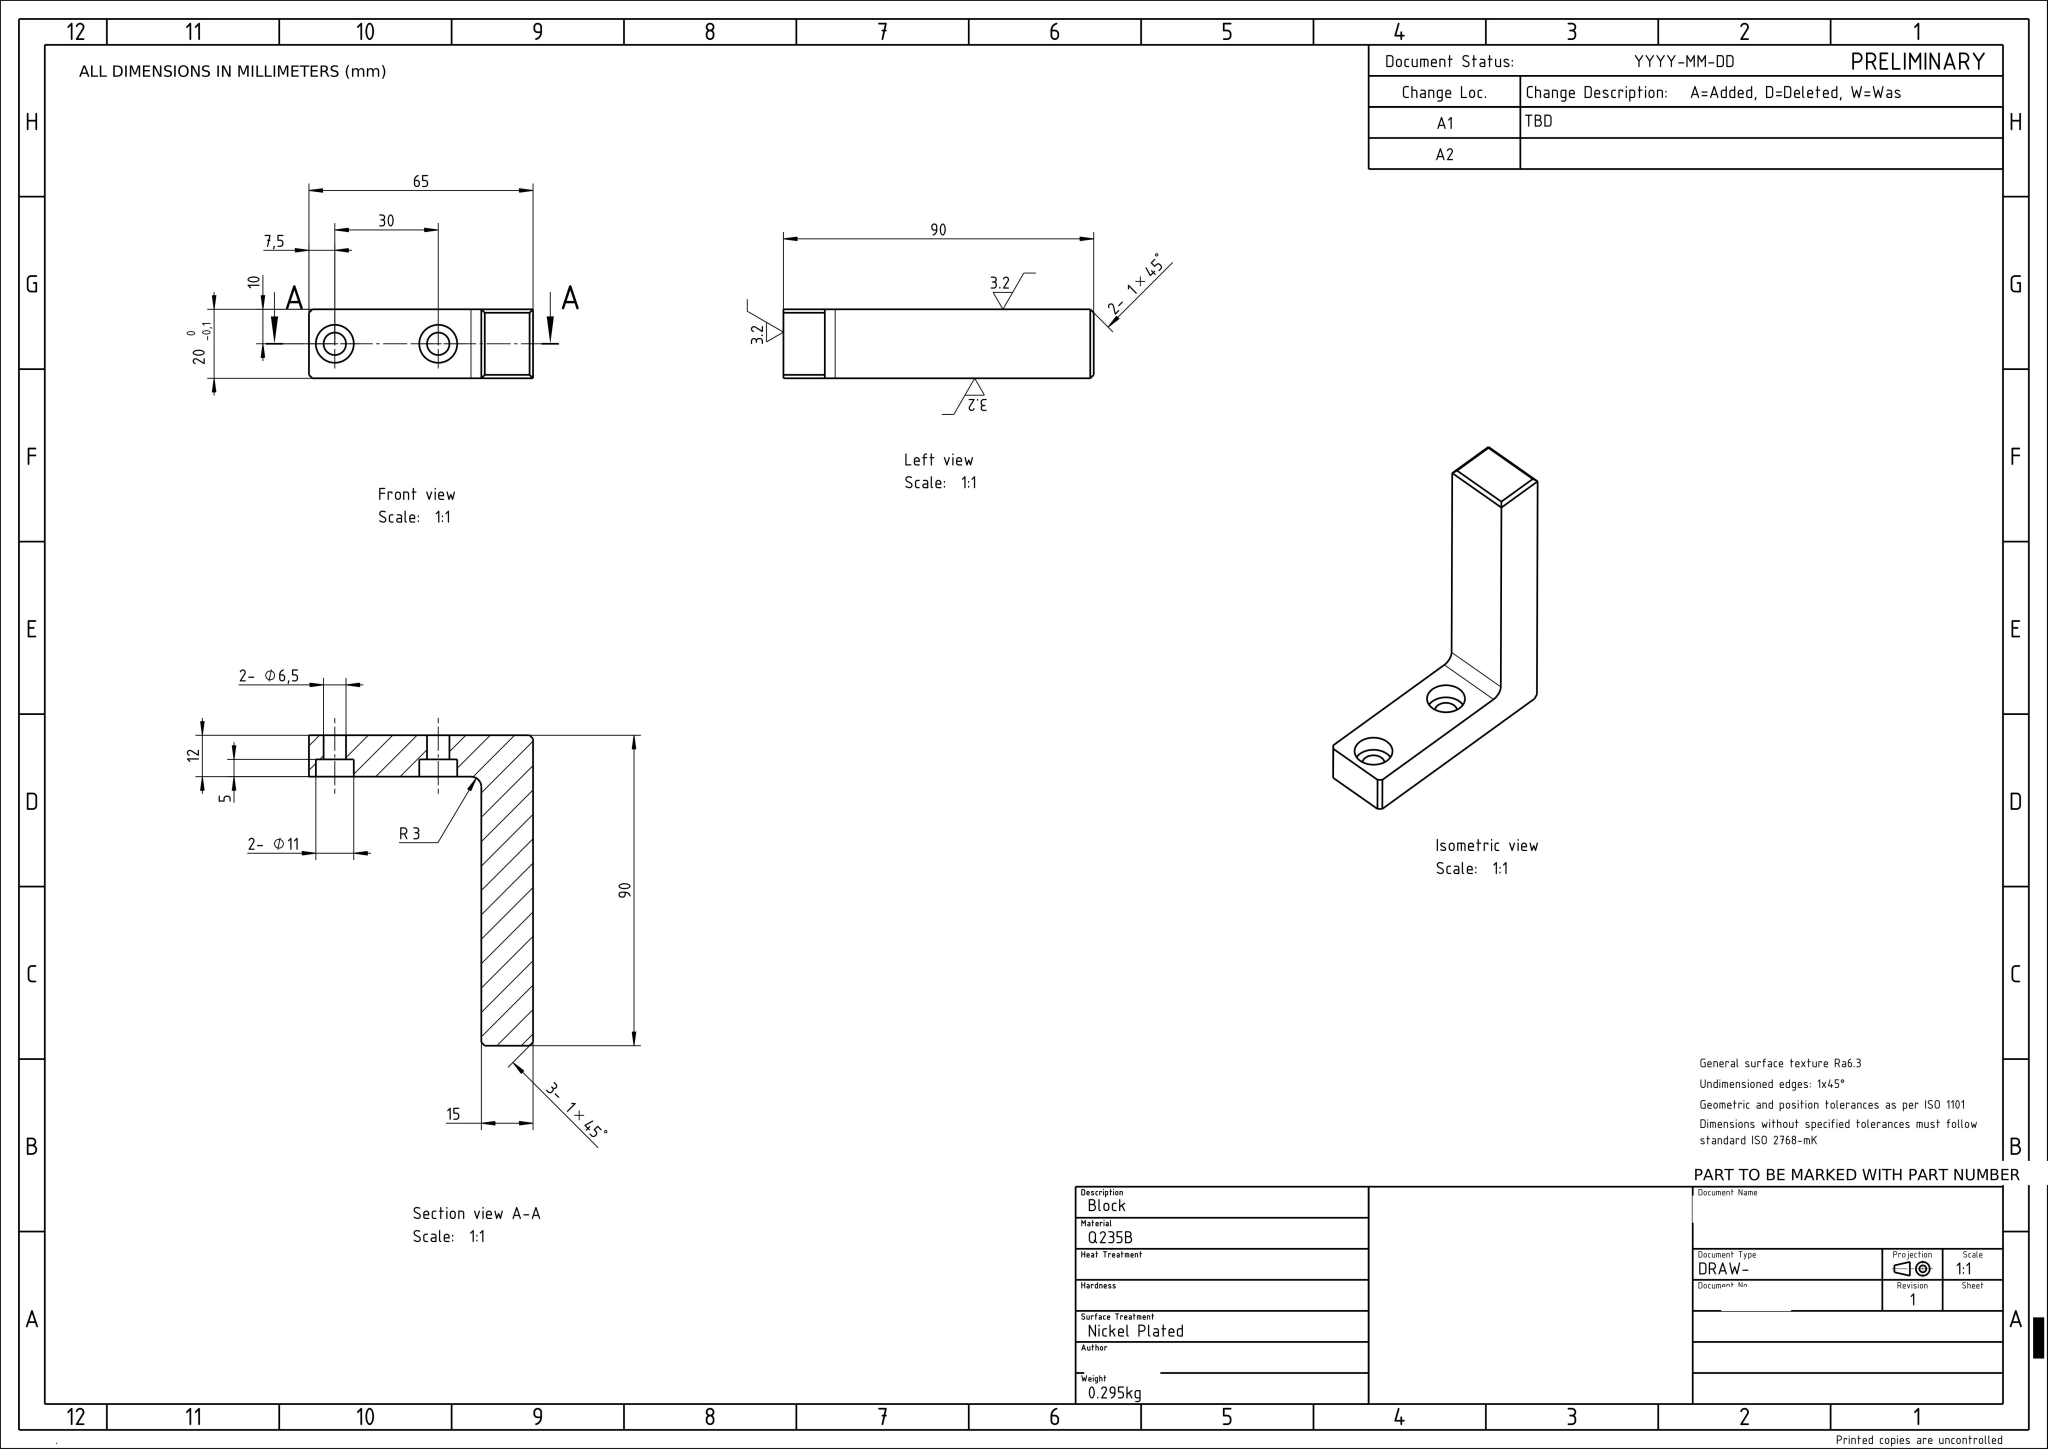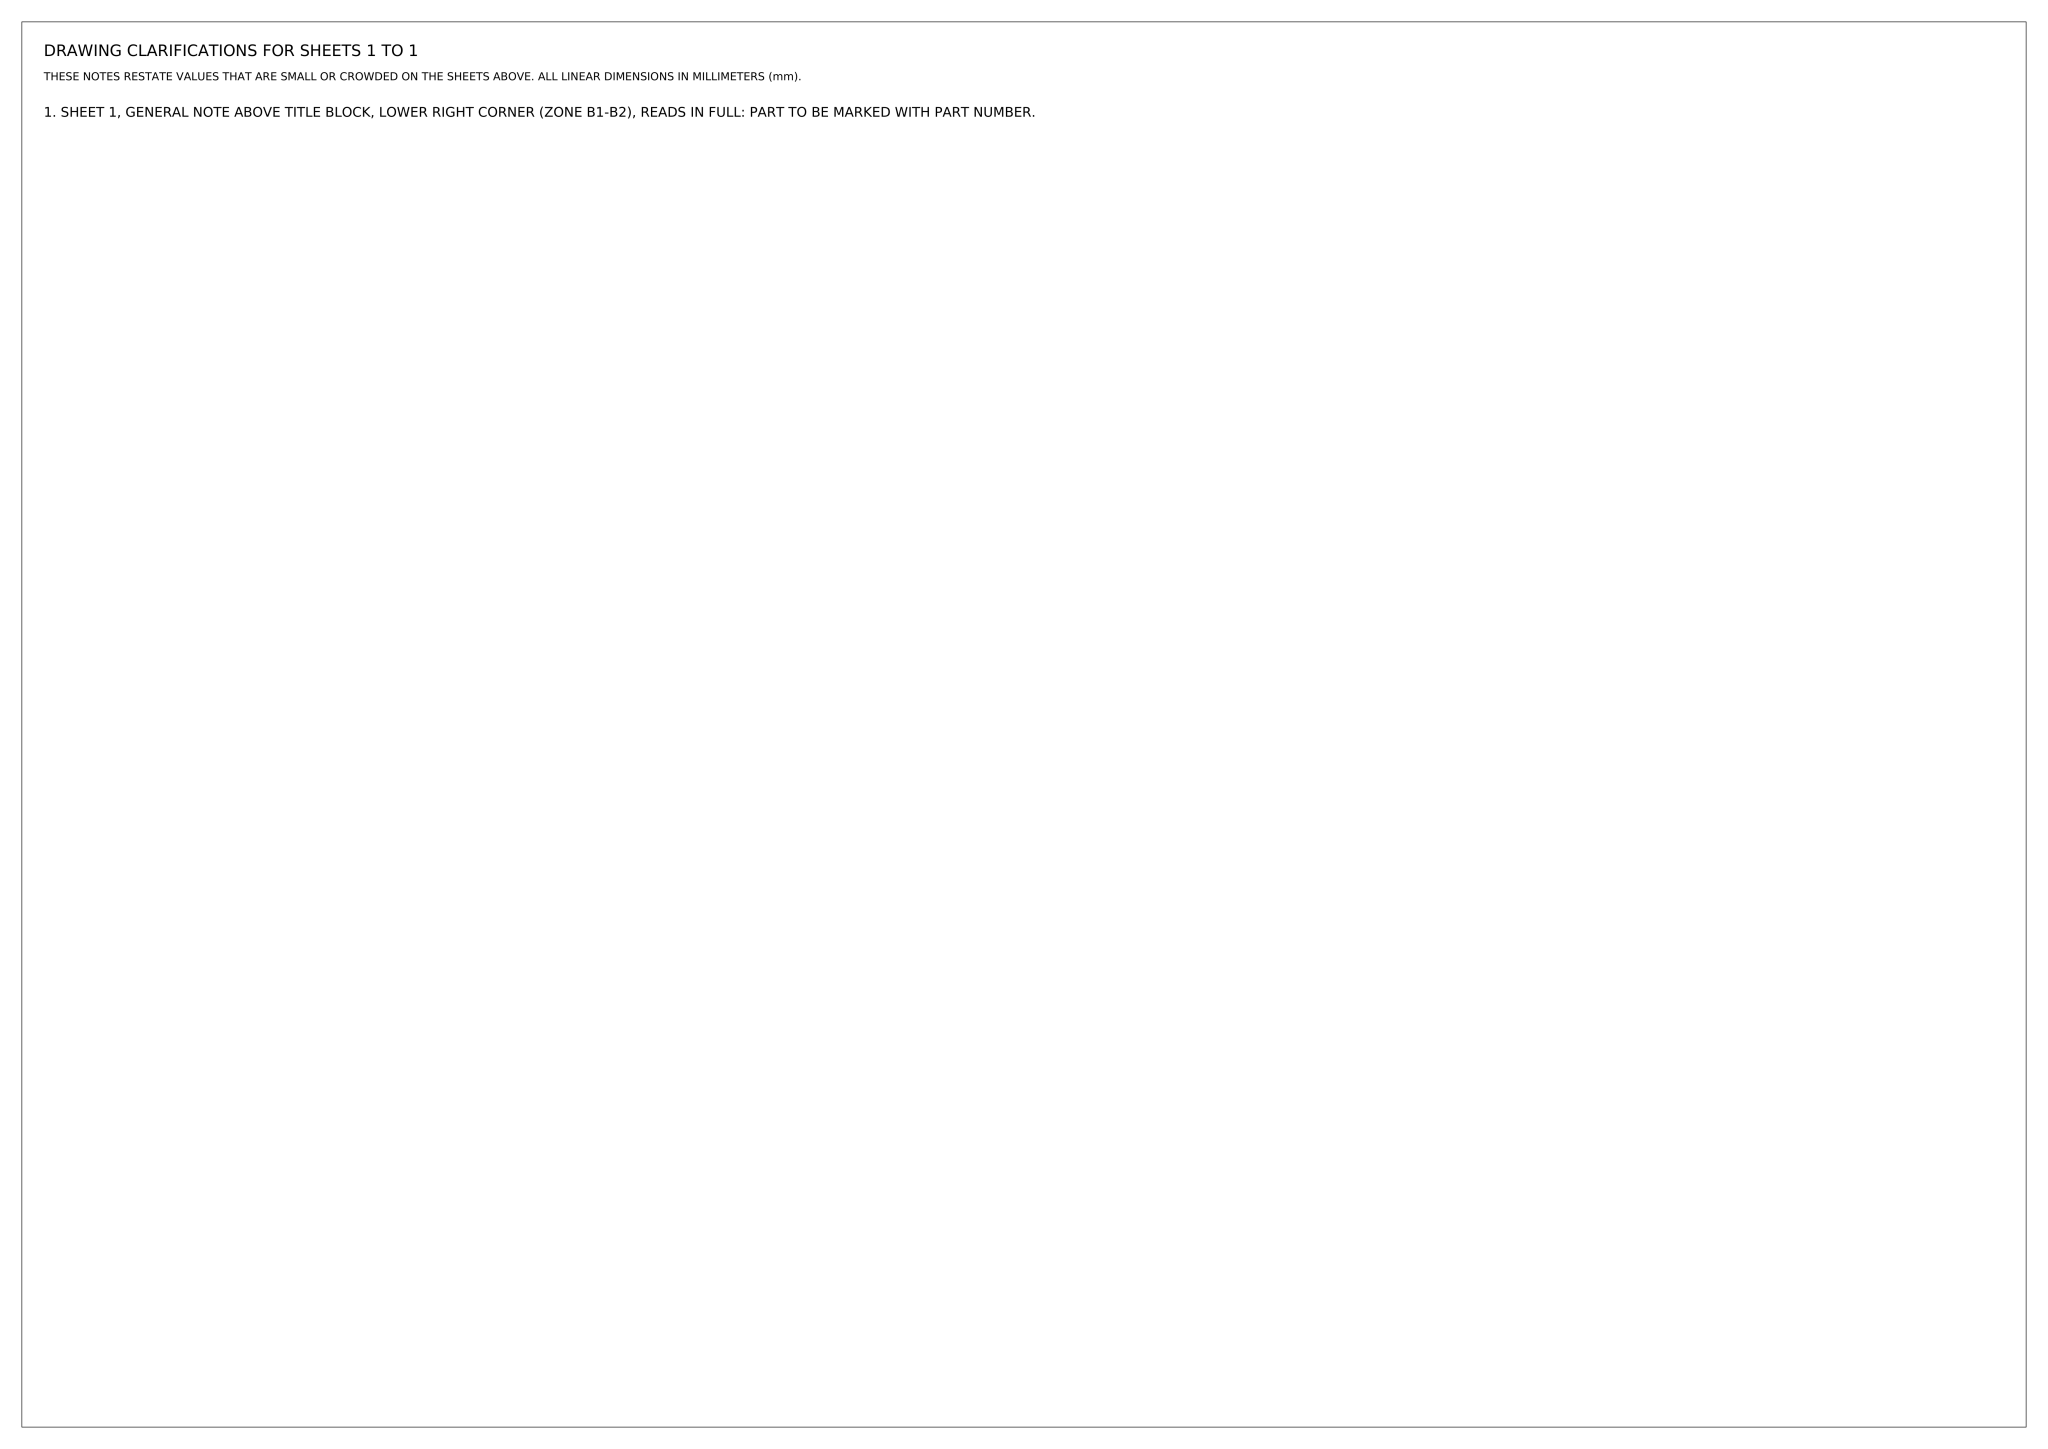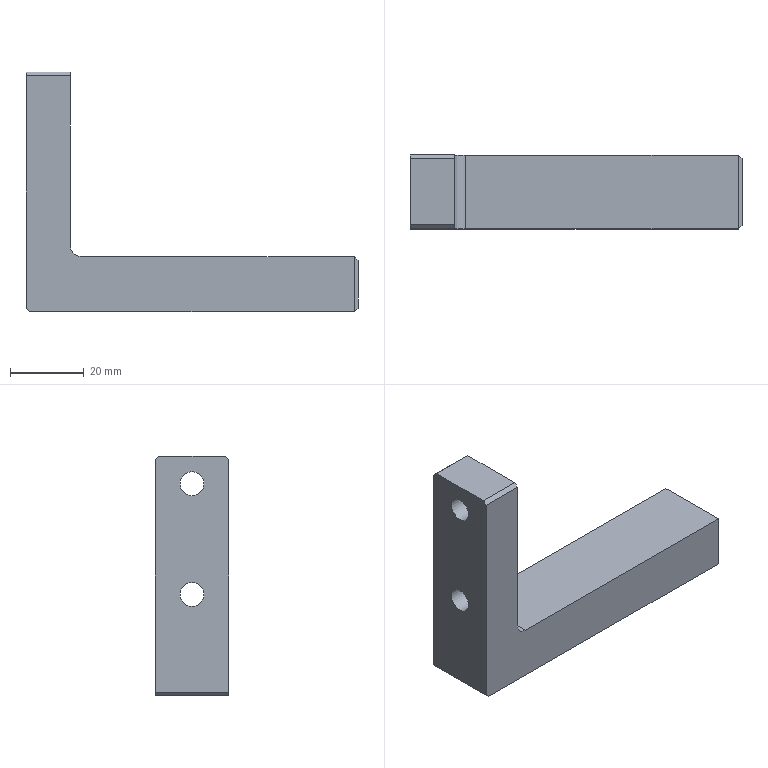Part | NX | mm | 1 solid | 22 faces | box 90 x 20 x 65 mm | volume 37568 mm3 | plane 17 | cylinder 5 | commonest cylinder face diameters 6.5 x2 11 x2 6 x1
STEP:
#1=CARTESIAN_POINT('',(0.,0.,0.));
#2=DIRECTION('',(0.,0.,1.));
#3=DIRECTION('',(1.,0.,0.));
#4=AXIS2_PLACEMENT_3D('',#1,#2,#3);
#5=(LENGTH_UNIT()NAMED_UNIT(*)SI_UNIT(.MILLI.,.METRE.));
#6=UNCERTAINTY_MEASURE_WITH_UNIT(LENGTH_MEASURE(0.00002),#5,'','');
#7=(NAMED_UNIT(*)PLANE_ANGLE_UNIT()SI_UNIT($,.RADIAN.));
#8=PLANE_ANGLE_MEASURE_WITH_UNIT(PLANE_ANGLE_MEASURE(0.01745),#7);
#9=DIMENSIONAL_EXPONENTS(0.,0.,0.,0.,0.,0.,0.);
#10=(CONVERSION_BASED_UNIT('',#8)NAMED_UNIT(#9)PLANE_ANGLE_UNIT());
#11=(NAMED_UNIT(*)SI_UNIT($,.STERADIAN.)SOLID_ANGLE_UNIT());
#12=(GEOMETRIC_REPRESENTATION_CONTEXT(3)GLOBAL_UNCERTAINTY_ASSIGNED_CONTEXT((#6))GLOBAL_UNIT_ASSIGNED_CONTEXT((#5,#10,#11))REPRESENTATION_CONTEXT('',''));
#13=SHAPE_REPRESENTATION('',(#4),#12);
#14=CARTESIAN_POINT('',(0.,-0.,54.25));
#15=VERTEX_POINT('',#14);
#16=CARTESIAN_POINT('',(0.,-0.,57.5));
#17=DIRECTION('',(1.,0.,0.));
#18=DIRECTION('',(0.,0.,-1.));
#19=AXIS2_PLACEMENT_3D('',#16,#17,#18);
#20=CIRCLE('',#19,3.25);
#21=EDGE_CURVE('',#15,#15,#20,.T.);
#22=ORIENTED_EDGE('',*,*,#21,.T.);
#23=EDGE_LOOP('',(#22));
#24=FACE_BOUND('',#23,.T.);
#25=CARTESIAN_POINT('',(0.,-0.,24.25));
#26=VERTEX_POINT('',#25);
#27=CARTESIAN_POINT('',(0.,-0.,27.5));
#28=DIRECTION('',(1.,0.,0.));
#29=DIRECTION('',(0.,0.,-1.));
#30=AXIS2_PLACEMENT_3D('',#27,#28,#29);
#31=CIRCLE('',#30,3.25);
#32=EDGE_CURVE('',#26,#26,#31,.T.);
#33=ORIENTED_EDGE('',*,*,#32,.T.);
#34=EDGE_LOOP('',(#33));
#35=FACE_BOUND('',#34,.T.);
#36=CARTESIAN_POINT('',(0.,10.,64.));
#37=VERTEX_POINT('',#36);
#38=CARTESIAN_POINT('',(0.,10.,1.));
#39=VERTEX_POINT('',#38);
#40=CARTESIAN_POINT('',(0.,10.,15.));
#41=DIRECTION('',(0.,0.,-1.));
#42=VECTOR('',#41,1.);
#43=LINE('',#40,#42);
#44=EDGE_CURVE('',#37,#39,#43,.T.);
#45=ORIENTED_EDGE('',*,*,#44,.T.);
#46=CARTESIAN_POINT('',(0.,-10.,1.));
#47=VERTEX_POINT('',#46);
#48=CARTESIAN_POINT('',(0.,10.,1.));
#49=DIRECTION('',(0.,-1.,0.));
#50=VECTOR('',#49,1.);
#51=LINE('',#48,#50);
#52=EDGE_CURVE('',#39,#47,#51,.T.);
#53=ORIENTED_EDGE('',*,*,#52,.T.);
#54=CARTESIAN_POINT('',(0.,-10.,64.));
#55=VERTEX_POINT('',#54);
#56=CARTESIAN_POINT('',(0.,-10.,15.));
#57=DIRECTION('',(0.,0.,-1.));
#58=VECTOR('',#57,1.);
#59=LINE('',#56,#58);
#60=EDGE_CURVE('',#55,#47,#59,.T.);
#61=ORIENTED_EDGE('',*,*,#60,.F.);
#62=CARTESIAN_POINT('',(0.,-9.,65.));
#63=VERTEX_POINT('',#62);
#64=CARTESIAN_POINT('',(0.,-9.,65.));
#65=DIRECTION('',(0.,0.7071,0.7071));
#66=VECTOR('',#65,1.);
#67=LINE('',#64,#66);
#68=EDGE_CURVE('',#55,#63,#67,.T.);
#69=ORIENTED_EDGE('',*,*,#68,.T.);
#70=CARTESIAN_POINT('',(0.,9.,65.));
#71=VERTEX_POINT('',#70);
#72=CARTESIAN_POINT('',(0.,-10.,65.));
#73=DIRECTION('',(0.,1.,0.));
#74=VECTOR('',#73,1.);
#75=LINE('',#72,#74);
#76=EDGE_CURVE('',#63,#71,#75,.T.);
#77=ORIENTED_EDGE('',*,*,#76,.T.);
#78=CARTESIAN_POINT('',(0.,10.,64.));
#79=DIRECTION('',(0.,0.7071,-0.7071));
#80=VECTOR('',#79,1.);
#81=LINE('',#78,#80);
#82=EDGE_CURVE('',#71,#37,#81,.T.);
#83=ORIENTED_EDGE('',*,*,#82,.T.);
#84=EDGE_LOOP('',(#45,#53,#61,#69,#77,#83));
#85=FACE_BOUND('',#84,.T.);
#86=CARTESIAN_POINT('',(0.,10.,15.));
#87=DIRECTION('',(1.,0.,0.));
#88=DIRECTION('',(0.,0.,-1.));
#89=AXIS2_PLACEMENT_3D('',#86,#87,#88);
#90=PLANE('',#89);
#91=ADVANCED_FACE('',(#24,#35,#85),#90,.F.);
#92=ORIENTED_EDGE('',*,*,#60,.T.);
#93=CARTESIAN_POINT('',(1.,-10.,0.));
#94=VERTEX_POINT('',#93);
#95=CARTESIAN_POINT('',(0.,-10.,1.));
#96=DIRECTION('',(0.7071,0.,-0.7071));
#97=VECTOR('',#96,1.);
#98=LINE('',#95,#97);
#99=EDGE_CURVE('',#47,#94,#98,.T.);
#100=ORIENTED_EDGE('',*,*,#99,.T.);
#101=CARTESIAN_POINT('',(89.,-10.,0.));
#102=VERTEX_POINT('',#101);
#103=CARTESIAN_POINT('',(0.,-10.,0.));
#104=DIRECTION('',(1.,0.,0.));
#105=VECTOR('',#104,1.);
#106=LINE('',#103,#105);
#107=EDGE_CURVE('',#94,#102,#106,.T.);
#108=ORIENTED_EDGE('',*,*,#107,.T.);
#109=CARTESIAN_POINT('',(89.,-10.,15.));
#110=VERTEX_POINT('',#109);
#111=CARTESIAN_POINT('',(89.,-10.,15.));
#112=DIRECTION('',(0.,0.,1.));
#113=VECTOR('',#112,1.);
#114=LINE('',#111,#113);
#115=EDGE_CURVE('',#102,#110,#114,.T.);
#116=ORIENTED_EDGE('',*,*,#115,.T.);
#117=CARTESIAN_POINT('',(15.,-10.,15.));
#118=VERTEX_POINT('',#117);
#119=CARTESIAN_POINT('',(0.,-10.,15.));
#120=DIRECTION('',(1.,0.,0.));
#121=VECTOR('',#120,1.);
#122=LINE('',#119,#121);
#123=EDGE_CURVE('',#118,#110,#122,.T.);
#124=ORIENTED_EDGE('',*,*,#123,.F.);
#125=CARTESIAN_POINT('',(12.,-10.,18.));
#126=VERTEX_POINT('',#125);
#127=CARTESIAN_POINT('',(15.,-10.,18.));
#128=DIRECTION('',(0.,1.,0.));
#129=DIRECTION('',(0.,0.,1.));
#130=AXIS2_PLACEMENT_3D('',#127,#128,#129);
#131=CIRCLE('',#130,3.);
#132=EDGE_CURVE('',#118,#126,#131,.T.);
#133=ORIENTED_EDGE('',*,*,#132,.T.);
#134=CARTESIAN_POINT('',(12.,-10.,64.));
#135=VERTEX_POINT('',#134);
#136=CARTESIAN_POINT('',(12.,-10.,15.));
#137=DIRECTION('',(0.,0.,1.));
#138=VECTOR('',#137,1.);
#139=LINE('',#136,#138);
#140=EDGE_CURVE('',#126,#135,#139,.T.);
#141=ORIENTED_EDGE('',*,*,#140,.T.);
#142=CARTESIAN_POINT('',(0.,-10.,64.));
#143=DIRECTION('',(-1.,0.,0.));
#144=VECTOR('',#143,1.);
#145=LINE('',#142,#144);
#146=EDGE_CURVE('',#135,#55,#145,.T.);
#147=ORIENTED_EDGE('',*,*,#146,.T.);
#148=EDGE_LOOP('',(#92,#100,#108,#116,#124,#133,#141,#147));
#149=FACE_OUTER_BOUND('',#148,.T.);
#150=CARTESIAN_POINT('',(0.,-10.,15.));
#151=DIRECTION('',(0.,1.,0.));
#152=DIRECTION('',(0.,0.,1.));
#153=AXIS2_PLACEMENT_3D('',#150,#151,#152);
#154=PLANE('',#153);
#155=ADVANCED_FACE('',(#149),#154,.F.);
#156=CARTESIAN_POINT('',(90.,9.,14.));
#157=VERTEX_POINT('',#156);
#158=CARTESIAN_POINT('',(90.,-9.,14.));
#159=VERTEX_POINT('',#158);
#160=CARTESIAN_POINT('',(90.,-10.,14.));
#161=DIRECTION('',(0.,-1.,0.));
#162=VECTOR('',#161,1.);
#163=LINE('',#160,#162);
#164=EDGE_CURVE('',#157,#159,#163,.T.);
#165=ORIENTED_EDGE('',*,*,#164,.T.);
#166=CARTESIAN_POINT('',(90.,-9.,1.));
#167=VERTEX_POINT('',#166);
#168=CARTESIAN_POINT('',(90.,-9.,15.));
#169=DIRECTION('',(0.,0.,-1.));
#170=VECTOR('',#169,1.);
#171=LINE('',#168,#170);
#172=EDGE_CURVE('',#159,#167,#171,.T.);
#173=ORIENTED_EDGE('',*,*,#172,.T.);
#174=CARTESIAN_POINT('',(90.,9.,1.));
#175=VERTEX_POINT('',#174);
#176=CARTESIAN_POINT('',(90.,-10.,1.));
#177=DIRECTION('',(0.,1.,0.));
#178=VECTOR('',#177,1.);
#179=LINE('',#176,#178);
#180=EDGE_CURVE('',#167,#175,#179,.T.);
#181=ORIENTED_EDGE('',*,*,#180,.T.);
#182=CARTESIAN_POINT('',(90.,9.,15.));
#183=DIRECTION('',(0.,0.,1.));
#184=VECTOR('',#183,1.);
#185=LINE('',#182,#184);
#186=EDGE_CURVE('',#175,#157,#185,.T.);
#187=ORIENTED_EDGE('',*,*,#186,.T.);
#188=EDGE_LOOP('',(#165,#173,#181,#187));
#189=FACE_OUTER_BOUND('',#188,.T.);
#190=CARTESIAN_POINT('',(90.,-10.,15.));
#191=DIRECTION('',(-1.,0.,0.));
#192=DIRECTION('',(0.,0.,1.));
#193=AXIS2_PLACEMENT_3D('',#190,#191,#192);
#194=PLANE('',#193);
#195=ADVANCED_FACE('',(#189),#194,.F.);
#196=CARTESIAN_POINT('',(89.,10.,0.));
#197=VERTEX_POINT('',#196);
#198=CARTESIAN_POINT('',(1.,10.,0.));
#199=VERTEX_POINT('',#198);
#200=CARTESIAN_POINT('',(90.,10.,0.));
#201=DIRECTION('',(-1.,0.,0.));
#202=VECTOR('',#201,1.);
#203=LINE('',#200,#202);
#204=EDGE_CURVE('',#197,#199,#203,.T.);
#205=ORIENTED_EDGE('',*,*,#204,.T.);
#206=CARTESIAN_POINT('',(0.,10.,1.));
#207=DIRECTION('',(-0.7071,0.,0.7071));
#208=VECTOR('',#207,1.);
#209=LINE('',#206,#208);
#210=EDGE_CURVE('',#199,#39,#209,.T.);
#211=ORIENTED_EDGE('',*,*,#210,.T.);
#212=ORIENTED_EDGE('',*,*,#44,.F.);
#213=CARTESIAN_POINT('',(12.,10.,64.));
#214=VERTEX_POINT('',#213);
#215=CARTESIAN_POINT('',(12.,10.,64.));
#216=DIRECTION('',(1.,0.,0.));
#217=VECTOR('',#216,1.);
#218=LINE('',#215,#217);
#219=EDGE_CURVE('',#37,#214,#218,.T.);
#220=ORIENTED_EDGE('',*,*,#219,.T.);
#221=CARTESIAN_POINT('',(12.,10.,18.));
#222=VERTEX_POINT('',#221);
#223=CARTESIAN_POINT('',(12.,10.,15.));
#224=DIRECTION('',(0.,0.,1.));
#225=VECTOR('',#224,1.);
#226=LINE('',#223,#225);
#227=EDGE_CURVE('',#222,#214,#226,.T.);
#228=ORIENTED_EDGE('',*,*,#227,.F.);
#229=CARTESIAN_POINT('',(15.,10.,15.));
#230=VERTEX_POINT('',#229);
#231=CARTESIAN_POINT('',(15.,10.,18.));
#232=DIRECTION('',(0.,-1.,0.));
#233=DIRECTION('',(0.,0.,-1.));
#234=AXIS2_PLACEMENT_3D('',#231,#232,#233);
#235=CIRCLE('',#234,3.);
#236=EDGE_CURVE('',#222,#230,#235,.T.);
#237=ORIENTED_EDGE('',*,*,#236,.T.);
#238=CARTESIAN_POINT('',(89.,10.,15.));
#239=VERTEX_POINT('',#238);
#240=CARTESIAN_POINT('',(90.,10.,15.));
#241=DIRECTION('',(-1.,0.,0.));
#242=VECTOR('',#241,1.);
#243=LINE('',#240,#242);
#244=EDGE_CURVE('',#239,#230,#243,.T.);
#245=ORIENTED_EDGE('',*,*,#244,.F.);
#246=CARTESIAN_POINT('',(89.,10.,15.));
#247=DIRECTION('',(0.,0.,-1.));
#248=VECTOR('',#247,1.);
#249=LINE('',#246,#248);
#250=EDGE_CURVE('',#239,#197,#249,.T.);
#251=ORIENTED_EDGE('',*,*,#250,.T.);
#252=EDGE_LOOP('',(#205,#211,#212,#220,#228,#237,#245,#251));
#253=FACE_OUTER_BOUND('',#252,.T.);
#254=CARTESIAN_POINT('',(90.,10.,15.));
#255=DIRECTION('',(0.,-1.,0.));
#256=DIRECTION('',(0.,0.,-1.));
#257=AXIS2_PLACEMENT_3D('',#254,#255,#256);
#258=PLANE('',#257);
#259=ADVANCED_FACE('',(#253),#258,.F.);
#260=ORIENTED_EDGE('',*,*,#123,.T.);
#261=CARTESIAN_POINT('',(89.,10.,15.));
#262=DIRECTION('',(0.,1.,0.));
#263=VECTOR('',#262,1.);
#264=LINE('',#261,#263);
#265=EDGE_CURVE('',#110,#239,#264,.T.);
#266=ORIENTED_EDGE('',*,*,#265,.T.);
#267=ORIENTED_EDGE('',*,*,#244,.T.);
#268=CARTESIAN_POINT('',(15.,-10.,15.));
#269=DIRECTION('',(0.,-1.,0.));
#270=VECTOR('',#269,1.);
#271=LINE('',#268,#270);
#272=EDGE_CURVE('',#230,#118,#271,.T.);
#273=ORIENTED_EDGE('',*,*,#272,.T.);
#274=EDGE_LOOP('',(#260,#266,#267,#273));
#275=FACE_OUTER_BOUND('',#274,.T.);
#276=CARTESIAN_POINT('',(0.,0.,15.));
#277=DIRECTION('',(0.,0.,1.));
#278=DIRECTION('',(1.,0.,0.));
#279=AXIS2_PLACEMENT_3D('',#276,#277,#278);
#280=PLANE('',#279);
#281=ADVANCED_FACE('',(#275),#280,.T.);
#282=ORIENTED_EDGE('',*,*,#107,.F.);
#283=CARTESIAN_POINT('',(1.,0.,0.));
#284=DIRECTION('',(0.,1.,0.));
#285=VECTOR('',#284,1.);
#286=LINE('',#283,#285);
#287=EDGE_CURVE('',#94,#199,#286,.T.);
#288=ORIENTED_EDGE('',*,*,#287,.T.);
#289=ORIENTED_EDGE('',*,*,#204,.F.);
#290=CARTESIAN_POINT('',(89.,0.,0.));
#291=DIRECTION('',(0.,-1.,0.));
#292=VECTOR('',#291,1.);
#293=LINE('',#290,#292);
#294=EDGE_CURVE('',#197,#102,#293,.T.);
#295=ORIENTED_EDGE('',*,*,#294,.T.);
#296=EDGE_LOOP('',(#282,#288,#289,#295));
#297=FACE_OUTER_BOUND('',#296,.T.);
#298=CARTESIAN_POINT('',(0.,0.,0.));
#299=DIRECTION('',(0.,0.,1.));
#300=DIRECTION('',(1.,0.,0.));
#301=AXIS2_PLACEMENT_3D('',#298,#299,#300);
#302=PLANE('',#301);
#303=ADVANCED_FACE('',(#297),#302,.F.);
#304=CARTESIAN_POINT('',(12.,-9.,65.));
#305=VERTEX_POINT('',#304);
#306=CARTESIAN_POINT('',(12.,9.,65.));
#307=VERTEX_POINT('',#306);
#308=CARTESIAN_POINT('',(12.,-10.,65.));
#309=DIRECTION('',(0.,1.,0.));
#310=VECTOR('',#309,1.);
#311=LINE('',#308,#310);
#312=EDGE_CURVE('',#305,#307,#311,.T.);
#313=ORIENTED_EDGE('',*,*,#312,.T.);
#314=CARTESIAN_POINT('',(0.,9.,65.));
#315=DIRECTION('',(-1.,0.,0.));
#316=VECTOR('',#315,1.);
#317=LINE('',#314,#316);
#318=EDGE_CURVE('',#307,#71,#317,.T.);
#319=ORIENTED_EDGE('',*,*,#318,.T.);
#320=ORIENTED_EDGE('',*,*,#76,.F.);
#321=CARTESIAN_POINT('',(12.,-9.,65.));
#322=DIRECTION('',(1.,0.,0.));
#323=VECTOR('',#322,1.);
#324=LINE('',#321,#323);
#325=EDGE_CURVE('',#63,#305,#324,.T.);
#326=ORIENTED_EDGE('',*,*,#325,.T.);
#327=EDGE_LOOP('',(#313,#319,#320,#326));
#328=FACE_OUTER_BOUND('',#327,.T.);
#329=CARTESIAN_POINT('',(0.,-10.,65.));
#330=DIRECTION('',(0.,0.,-1.));
#331=DIRECTION('',(0.,1.,0.));
#332=AXIS2_PLACEMENT_3D('',#329,#330,#331);
#333=PLANE('',#332);
#334=ADVANCED_FACE('',(#328),#333,.F.);
#335=CARTESIAN_POINT('',(12.,-0.,63.));
#336=VERTEX_POINT('',#335);
#337=CARTESIAN_POINT('',(12.,-0.,57.5));
#338=DIRECTION('',(-1.,0.,0.));
#339=DIRECTION('',(0.,0.,1.));
#340=AXIS2_PLACEMENT_3D('',#337,#338,#339);
#341=CIRCLE('',#340,5.5);
#342=EDGE_CURVE('',#336,#336,#341,.T.);
#343=ORIENTED_EDGE('',*,*,#342,.T.);
#344=EDGE_LOOP('',(#343));
#345=FACE_BOUND('',#344,.T.);
#346=CARTESIAN_POINT('',(12.,-0.,33.));
#347=VERTEX_POINT('',#346);
#348=CARTESIAN_POINT('',(12.,-0.,27.5));
#349=DIRECTION('',(-1.,0.,0.));
#350=DIRECTION('',(0.,0.,1.));
#351=AXIS2_PLACEMENT_3D('',#348,#349,#350);
#352=CIRCLE('',#351,5.5);
#353=EDGE_CURVE('',#347,#347,#352,.T.);
#354=ORIENTED_EDGE('',*,*,#353,.T.);
#355=EDGE_LOOP('',(#354));
#356=FACE_BOUND('',#355,.T.);
#357=ORIENTED_EDGE('',*,*,#227,.T.);
#358=CARTESIAN_POINT('',(12.,24.5,49.5));
#359=DIRECTION('',(0.,-0.7071,0.7071));
#360=VECTOR('',#359,1.);
#361=LINE('',#358,#360);
#362=EDGE_CURVE('',#214,#307,#361,.T.);
#363=ORIENTED_EDGE('',*,*,#362,.T.);
#364=ORIENTED_EDGE('',*,*,#312,.F.);
#365=CARTESIAN_POINT('',(12.,-34.5,39.5));
#366=DIRECTION('',(0.,-0.7071,-0.7071));
#367=VECTOR('',#366,1.);
#368=LINE('',#365,#367);
#369=EDGE_CURVE('',#305,#135,#368,.T.);
#370=ORIENTED_EDGE('',*,*,#369,.T.);
#371=ORIENTED_EDGE('',*,*,#140,.F.);
#372=CARTESIAN_POINT('',(12.,10.,18.));
#373=DIRECTION('',(0.,1.,0.));
#374=VECTOR('',#373,1.);
#375=LINE('',#372,#374);
#376=EDGE_CURVE('',#126,#222,#375,.T.);
#377=ORIENTED_EDGE('',*,*,#376,.T.);
#378=EDGE_LOOP('',(#357,#363,#364,#370,#371,#377));
#379=FACE_BOUND('',#378,.T.);
#380=CARTESIAN_POINT('',(12.,-10.,15.));
#381=DIRECTION('',(1.,0.,0.));
#382=DIRECTION('',(0.,0.,-1.));
#383=AXIS2_PLACEMENT_3D('',#380,#381,#382);
#384=PLANE('',#383);
#385=ADVANCED_FACE('',(#345,#356,#379),#384,.T.);
#386=CARTESIAN_POINT('',(7.,-0.,30.75));
#387=VERTEX_POINT('',#386);
#388=CARTESIAN_POINT('',(7.,-0.,27.5));
#389=DIRECTION('',(1.,0.,0.));
#390=DIRECTION('',(0.,0.,1.));
#391=AXIS2_PLACEMENT_3D('',#388,#389,#390);
#392=CIRCLE('',#391,3.25);
#393=EDGE_CURVE('',#387,#387,#392,.T.);
#394=ORIENTED_EDGE('',*,*,#393,.T.);
#395=EDGE_LOOP('',(#394));
#396=FACE_BOUND('',#395,.T.);
#397=ORIENTED_EDGE('',*,*,#32,.F.);
#398=EDGE_LOOP('',(#397));
#399=FACE_BOUND('',#398,.T.);
#400=CARTESIAN_POINT('',(-16.841,-0.,27.5));
#401=DIRECTION('',(-1.,0.,0.));
#402=DIRECTION('',(0.,0.,1.));
#403=AXIS2_PLACEMENT_3D('',#400,#401,#402);
#404=CYLINDRICAL_SURFACE('',#403,3.25);
#405=ADVANCED_FACE('',(#396,#399),#404,.F.);
#406=ORIENTED_EDGE('',*,*,#393,.F.);
#407=EDGE_LOOP('',(#406));
#408=FACE_BOUND('',#407,.T.);
#409=CARTESIAN_POINT('',(7.,-0.,33.));
#410=VERTEX_POINT('',#409);
#411=CARTESIAN_POINT('',(7.,-0.,27.5));
#412=DIRECTION('',(1.,0.,0.));
#413=DIRECTION('',(0.,0.,1.));
#414=AXIS2_PLACEMENT_3D('',#411,#412,#413);
#415=CIRCLE('',#414,5.5);
#416=EDGE_CURVE('',#410,#410,#415,.T.);
#417=ORIENTED_EDGE('',*,*,#416,.T.);
#418=EDGE_LOOP('',(#417));
#419=FACE_BOUND('',#418,.T.);
#420=CARTESIAN_POINT('',(7.,-0.,27.5));
#421=DIRECTION('',(-1.,0.,0.));
#422=DIRECTION('',(0.,0.,1.));
#423=AXIS2_PLACEMENT_3D('',#420,#421,#422);
#424=PLANE('',#423);
#425=ADVANCED_FACE('',(#408,#419),#424,.F.);
#426=ORIENTED_EDGE('',*,*,#416,.F.);
#427=EDGE_LOOP('',(#426));
#428=FACE_BOUND('',#427,.T.);
#429=ORIENTED_EDGE('',*,*,#353,.F.);
#430=EDGE_LOOP('',(#429));
#431=FACE_BOUND('',#430,.T.);
#432=CARTESIAN_POINT('',(12.,-0.,27.5));
#433=DIRECTION('',(-1.,0.,0.));
#434=DIRECTION('',(0.,0.,1.));
#435=AXIS2_PLACEMENT_3D('',#432,#433,#434);
#436=CYLINDRICAL_SURFACE('',#435,5.5);
#437=ADVANCED_FACE('',(#428,#431),#436,.F.);
#438=CARTESIAN_POINT('',(7.,-0.,60.75));
#439=VERTEX_POINT('',#438);
#440=CARTESIAN_POINT('',(7.,-0.,57.5));
#441=DIRECTION('',(1.,0.,0.));
#442=DIRECTION('',(0.,0.,1.));
#443=AXIS2_PLACEMENT_3D('',#440,#441,#442);
#444=CIRCLE('',#443,3.25);
#445=EDGE_CURVE('',#439,#439,#444,.T.);
#446=ORIENTED_EDGE('',*,*,#445,.T.);
#447=EDGE_LOOP('',(#446));
#448=FACE_BOUND('',#447,.T.);
#449=ORIENTED_EDGE('',*,*,#21,.F.);
#450=EDGE_LOOP('',(#449));
#451=FACE_BOUND('',#450,.T.);
#452=CARTESIAN_POINT('',(-11.783,-0.,57.5));
#453=DIRECTION('',(-1.,0.,0.));
#454=DIRECTION('',(0.,0.,1.));
#455=AXIS2_PLACEMENT_3D('',#452,#453,#454);
#456=CYLINDRICAL_SURFACE('',#455,3.25);
#457=ADVANCED_FACE('',(#448,#451),#456,.F.);
#458=ORIENTED_EDGE('',*,*,#445,.F.);
#459=EDGE_LOOP('',(#458));
#460=FACE_BOUND('',#459,.T.);
#461=CARTESIAN_POINT('',(7.,-0.,63.));
#462=VERTEX_POINT('',#461);
#463=CARTESIAN_POINT('',(7.,-0.,57.5));
#464=DIRECTION('',(1.,0.,0.));
#465=DIRECTION('',(0.,0.,1.));
#466=AXIS2_PLACEMENT_3D('',#463,#464,#465);
#467=CIRCLE('',#466,5.5);
#468=EDGE_CURVE('',#462,#462,#467,.T.);
#469=ORIENTED_EDGE('',*,*,#468,.T.);
#470=EDGE_LOOP('',(#469));
#471=FACE_BOUND('',#470,.T.);
#472=CARTESIAN_POINT('',(7.,-0.,57.5));
#473=DIRECTION('',(-1.,0.,0.));
#474=DIRECTION('',(0.,0.,1.));
#475=AXIS2_PLACEMENT_3D('',#472,#473,#474);
#476=PLANE('',#475);
#477=ADVANCED_FACE('',(#460,#471),#476,.F.);
#478=ORIENTED_EDGE('',*,*,#468,.F.);
#479=EDGE_LOOP('',(#478));
#480=FACE_BOUND('',#479,.T.);
#481=ORIENTED_EDGE('',*,*,#342,.F.);
#482=EDGE_LOOP('',(#481));
#483=FACE_BOUND('',#482,.T.);
#484=CARTESIAN_POINT('',(12.,-0.,57.5));
#485=DIRECTION('',(-1.,0.,0.));
#486=DIRECTION('',(0.,0.,1.));
#487=AXIS2_PLACEMENT_3D('',#484,#485,#486);
#488=CYLINDRICAL_SURFACE('',#487,5.5);
#489=ADVANCED_FACE('',(#480,#483),#488,.F.);
#490=ORIENTED_EDGE('',*,*,#132,.F.);
#491=ORIENTED_EDGE('',*,*,#272,.F.);
#492=ORIENTED_EDGE('',*,*,#236,.F.);
#493=ORIENTED_EDGE('',*,*,#376,.F.);
#494=EDGE_LOOP('',(#490,#491,#492,#493));
#495=FACE_OUTER_BOUND('',#494,.T.);
#496=CARTESIAN_POINT('',(15.,-10.,18.));
#497=DIRECTION('',(0.,-1.,0.));
#498=DIRECTION('',(0.,0.,-1.));
#499=AXIS2_PLACEMENT_3D('',#496,#497,#498);
#500=CYLINDRICAL_SURFACE('',#499,3.);
#501=ADVANCED_FACE('',(#495),#500,.F.);
#502=ORIENTED_EDGE('',*,*,#210,.F.);
#503=ORIENTED_EDGE('',*,*,#287,.F.);
#504=ORIENTED_EDGE('',*,*,#99,.F.);
#505=ORIENTED_EDGE('',*,*,#52,.F.);
#506=EDGE_LOOP('',(#502,#503,#504,#505));
#507=FACE_OUTER_BOUND('',#506,.T.);
#508=CARTESIAN_POINT('',(0.,10.,1.));
#509=DIRECTION('',(0.7071,0.,0.7071));
#510=DIRECTION('',(0.,-1.,0.));
#511=AXIS2_PLACEMENT_3D('',#508,#509,#510);
#512=PLANE('',#511);
#513=ADVANCED_FACE('',(#507),#512,.F.);
#514=CARTESIAN_POINT('',(96.333,2.667,7.333));
#515=DIRECTION('',(0.5774,-0.5774,0.5774));
#516=VECTOR('',#515,1.);
#517=LINE('',#514,#516);
#518=EDGE_CURVE('',#197,#175,#517,.T.);
#519=ORIENTED_EDGE('',*,*,#518,.F.);
#520=ORIENTED_EDGE('',*,*,#250,.F.);
#521=CARTESIAN_POINT('',(89.,10.,15.));
#522=DIRECTION('',(-0.5774,0.5774,0.5774));
#523=VECTOR('',#522,1.);
#524=LINE('',#521,#523);
#525=EDGE_CURVE('',#157,#239,#524,.T.);
#526=ORIENTED_EDGE('',*,*,#525,.F.);
#527=ORIENTED_EDGE('',*,*,#186,.F.);
#528=EDGE_LOOP('',(#519,#520,#526,#527));
#529=FACE_OUTER_BOUND('',#528,.T.);
#530=CARTESIAN_POINT('',(89.,10.,15.));
#531=DIRECTION('',(-0.7071,-0.7071,0.));
#532=DIRECTION('',(0.,0.,-1.));
#533=AXIS2_PLACEMENT_3D('',#530,#531,#532);
#534=PLANE('',#533);
#535=ADVANCED_FACE('',(#529),#534,.F.);
#536=ORIENTED_EDGE('',*,*,#525,.T.);
#537=ORIENTED_EDGE('',*,*,#265,.F.);
#538=CARTESIAN_POINT('',(92.333,-6.667,11.667));
#539=DIRECTION('',(-0.5774,-0.5774,0.5774));
#540=VECTOR('',#539,1.);
#541=LINE('',#538,#540);
#542=EDGE_CURVE('',#159,#110,#541,.T.);
#543=ORIENTED_EDGE('',*,*,#542,.F.);
#544=ORIENTED_EDGE('',*,*,#164,.F.);
#545=EDGE_LOOP('',(#536,#537,#543,#544));
#546=FACE_OUTER_BOUND('',#545,.T.);
#547=CARTESIAN_POINT('',(89.,0.,15.));
#548=DIRECTION('',(0.7071,0.,0.7071));
#549=DIRECTION('',(0.,-1.,0.));
#550=AXIS2_PLACEMENT_3D('',#547,#548,#549);
#551=PLANE('',#550);
#552=ADVANCED_FACE('',(#546),#551,.T.);
#553=ORIENTED_EDGE('',*,*,#518,.T.);
#554=ORIENTED_EDGE('',*,*,#180,.F.);
#555=CARTESIAN_POINT('',(89.667,-9.333,0.6667));
#556=DIRECTION('',(0.5774,0.5774,0.5774));
#557=VECTOR('',#556,1.);
#558=LINE('',#555,#557);
#559=EDGE_CURVE('',#102,#167,#558,.T.);
#560=ORIENTED_EDGE('',*,*,#559,.F.);
#561=ORIENTED_EDGE('',*,*,#294,.F.);
#562=EDGE_LOOP('',(#553,#554,#560,#561));
#563=FACE_OUTER_BOUND('',#562,.T.);
#564=CARTESIAN_POINT('',(90.,-10.,1.));
#565=DIRECTION('',(-0.7071,0.,0.7071));
#566=DIRECTION('',(0.,1.,0.));
#567=AXIS2_PLACEMENT_3D('',#564,#565,#566);
#568=PLANE('',#567);
#569=ADVANCED_FACE('',(#563),#568,.F.);
#570=ORIENTED_EDGE('',*,*,#542,.T.);
#571=ORIENTED_EDGE('',*,*,#115,.F.);
#572=ORIENTED_EDGE('',*,*,#559,.T.);
#573=ORIENTED_EDGE('',*,*,#172,.F.);
#574=EDGE_LOOP('',(#570,#571,#572,#573));
#575=FACE_OUTER_BOUND('',#574,.T.);
#576=CARTESIAN_POINT('',(90.,-9.,15.));
#577=DIRECTION('',(-0.7071,0.7071,0.));
#578=DIRECTION('',(0.,0.,-1.));
#579=AXIS2_PLACEMENT_3D('',#576,#577,#578);
#580=PLANE('',#579);
#581=ADVANCED_FACE('',(#575),#580,.F.);
#582=ORIENTED_EDGE('',*,*,#82,.F.);
#583=ORIENTED_EDGE('',*,*,#318,.F.);
#584=ORIENTED_EDGE('',*,*,#362,.F.);
#585=ORIENTED_EDGE('',*,*,#219,.F.);
#586=EDGE_LOOP('',(#582,#583,#584,#585));
#587=FACE_OUTER_BOUND('',#586,.T.);
#588=CARTESIAN_POINT('',(90.,10.,64.));
#589=DIRECTION('',(0.,-0.7071,-0.7071));
#590=DIRECTION('',(1.,0.,0.));
#591=AXIS2_PLACEMENT_3D('',#588,#589,#590);
#592=PLANE('',#591);
#593=ADVANCED_FACE('',(#587),#592,.F.);
#594=ORIENTED_EDGE('',*,*,#68,.F.);
#595=ORIENTED_EDGE('',*,*,#146,.F.);
#596=ORIENTED_EDGE('',*,*,#369,.F.);
#597=ORIENTED_EDGE('',*,*,#325,.F.);
#598=EDGE_LOOP('',(#594,#595,#596,#597));
#599=FACE_OUTER_BOUND('',#598,.T.);
#600=CARTESIAN_POINT('',(0.,-9.,65.));
#601=DIRECTION('',(0.,0.7071,-0.7071));
#602=DIRECTION('',(1.,0.,0.));
#603=AXIS2_PLACEMENT_3D('',#600,#601,#602);
#604=PLANE('',#603);
#605=ADVANCED_FACE('',(#599),#604,.F.);
#606=CLOSED_SHELL('',(#91,#155,#195,#259,#281,#303,#334,#385,#405,#425,#437,#457,#477,#489,#501,#513,#535,#552,#569,#581,#593,#605));
#607=MANIFOLD_SOLID_BREP('',#606);
#608=ADVANCED_BREP_SHAPE_REPRESENTATION('',(#607),#12);
#609=SHAPE_REPRESENTATION_RELATIONSHIP('','',#13,#608);
#610=PRESENTATION_LAYER_ASSIGNMENT('','',(#607));
#611=COLOUR_RGB('',0.4,0.8,1.);
#612=FILL_AREA_STYLE_COLOUR('',#611);
#613=FILL_AREA_STYLE('',(#612));
#614=SURFACE_STYLE_FILL_AREA(#613);
#615=SURFACE_SIDE_STYLE('',(#614));
#616=SURFACE_STYLE_USAGE(.BOTH.,#615);
#617=PRESENTATION_STYLE_ASSIGNMENT((#616));
#618=STYLED_ITEM('',(#617),#607);
#619=MECHANICAL_DESIGN_GEOMETRIC_PRESENTATION_REPRESENTATION('',(#618),#12);